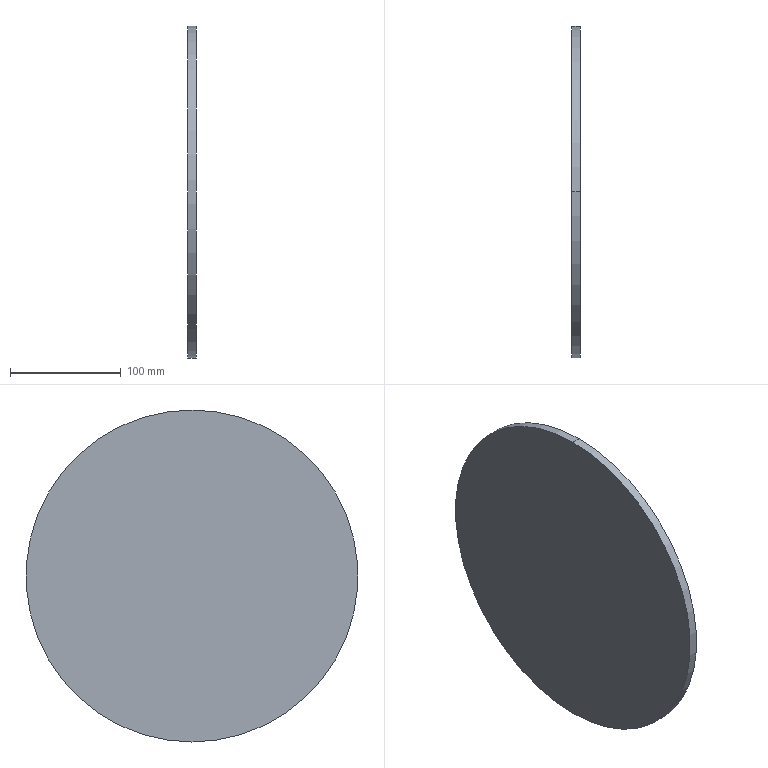Component | SolidWorks | JF21-80.1-1-3(_)-1-SOLID2-1 | 1 solid | 4 faces | box 8 x 300 x 300 mm | volume 565487 mm3 | cylinder 2 | plane 2 | commonest cylinder face diameters 300 x2
STEP:
#1=CARTESIAN_POINT('',(15.433,-39.37,42.126));
#2=VERTEX_POINT('',#1);
#3=CARTESIAN_POINT('',(15.433,-39.37,30.315));
#4=VERTEX_POINT('',#3);
#5=CARTESIAN_POINT('',(15.433,-39.37,36.22));
#6=DIRECTION('',(-1.,0.,0.));
#7=DIRECTION('',(0.,0.,1.));
#8=AXIS2_PLACEMENT_3D('',#5,#6,#7);
#9=CIRCLE('',#8,5.906);
#10=EDGE_CURVE('',#2,#4,#9,.T.);
#11=ORIENTED_EDGE('',*,*,#10,.F.);
#12=CARTESIAN_POINT('',(15.748,-39.37,42.126));
#13=VERTEX_POINT('',#12);
#14=CARTESIAN_POINT('',(15.433,-39.37,42.126));
#15=DIRECTION('',(-1.,0.,0.));
#16=VECTOR('',#15,39.37);
#17=LINE('',#14,#16);
#18=EDGE_CURVE('',#13,#2,#17,.T.);
#19=ORIENTED_EDGE('',*,*,#18,.F.);
#20=CARTESIAN_POINT('',(15.748,-39.37,30.315));
#21=VERTEX_POINT('',#20);
#22=CARTESIAN_POINT('',(15.748,-39.37,36.22));
#23=DIRECTION('',(-1.,0.,0.));
#24=DIRECTION('',(0.,0.,1.));
#25=AXIS2_PLACEMENT_3D('',#22,#23,#24);
#26=CIRCLE('',#25,5.906);
#27=EDGE_CURVE('',#13,#21,#26,.T.);
#28=ORIENTED_EDGE('',*,*,#27,.T.);
#29=CARTESIAN_POINT('',(15.433,-39.37,30.315));
#30=DIRECTION('',(-1.,0.,0.));
#31=VECTOR('',#30,39.37);
#32=LINE('',#29,#31);
#33=EDGE_CURVE('',#21,#4,#32,.T.);
#34=ORIENTED_EDGE('',*,*,#33,.T.);
#35=EDGE_LOOP('',(#11,#19,#28,#34));
#36=FACE_OUTER_BOUND('',#35,.T.);
#37=CARTESIAN_POINT('',(15.433,-39.37,36.22));
#38=DIRECTION('',(1.,0.,0.));
#39=DIRECTION('',(0.,0.,1.));
#40=AXIS2_PLACEMENT_3D('',#37,#38,#39);
#41=CYLINDRICAL_SURFACE('',#40,5.906);
#42=ADVANCED_FACE('',(#36),#41,.T.);
#43=ORIENTED_EDGE('',*,*,#18,.T.);
#44=CARTESIAN_POINT('',(15.433,-39.37,36.22));
#45=DIRECTION('',(-1.,0.,0.));
#46=DIRECTION('',(0.,0.,1.));
#47=AXIS2_PLACEMENT_3D('',#44,#45,#46);
#48=CIRCLE('',#47,5.906);
#49=EDGE_CURVE('',#4,#2,#48,.T.);
#50=ORIENTED_EDGE('',*,*,#49,.F.);
#51=ORIENTED_EDGE('',*,*,#33,.F.);
#52=CARTESIAN_POINT('',(15.748,-39.37,36.22));
#53=DIRECTION('',(-1.,0.,0.));
#54=DIRECTION('',(0.,0.,1.));
#55=AXIS2_PLACEMENT_3D('',#52,#53,#54);
#56=CIRCLE('',#55,5.906);
#57=EDGE_CURVE('',#21,#13,#56,.T.);
#58=ORIENTED_EDGE('',*,*,#57,.T.);
#59=EDGE_LOOP('',(#43,#50,#51,#58));
#60=FACE_OUTER_BOUND('',#59,.T.);
#61=CARTESIAN_POINT('',(15.433,-39.37,36.22));
#62=DIRECTION('',(1.,0.,0.));
#63=DIRECTION('',(0.,0.,1.));
#64=AXIS2_PLACEMENT_3D('',#61,#62,#63);
#65=CYLINDRICAL_SURFACE('',#64,5.906);
#66=ADVANCED_FACE('',(#60),#65,.T.);
#67=ORIENTED_EDGE('',*,*,#49,.T.);
#68=ORIENTED_EDGE('',*,*,#10,.T.);
#69=EDGE_LOOP('',(#67,#68));
#70=FACE_OUTER_BOUND('',#69,.T.);
#71=CARTESIAN_POINT('',(15.433,-39.37,36.22));
#72=DIRECTION('',(-1.,0.,0.));
#73=DIRECTION('',(0.,0.,-1.));
#74=AXIS2_PLACEMENT_3D('',#71,#72,#73);
#75=PLANE('',#74);
#76=ADVANCED_FACE('',(#70),#75,.T.);
#77=ORIENTED_EDGE('',*,*,#57,.F.);
#78=ORIENTED_EDGE('',*,*,#27,.F.);
#79=EDGE_LOOP('',(#77,#78));
#80=FACE_OUTER_BOUND('',#79,.T.);
#81=CARTESIAN_POINT('',(15.748,-39.37,36.22));
#82=DIRECTION('',(-1.,0.,0.));
#83=DIRECTION('',(0.,0.,-1.));
#84=AXIS2_PLACEMENT_3D('',#81,#82,#83);
#85=PLANE('',#84);
#86=ADVANCED_FACE('',(#80),#85,.F.);
#87=CLOSED_SHELL('',(#42,#66,#76,#86));
#88=MANIFOLD_SOLID_BREP('',#87);
#89=CARTESIAN_POINT('',(0.,0.,0.));
#90=DIRECTION('',(0.,0.,1.));
#91=DIRECTION('',(1.,0.,0.));
#92=AXIS2_PLACEMENT_3D('',#89,#90,#91);
#93=(LENGTH_UNIT()NAMED_UNIT(*)SI_UNIT($,.METRE.));
#94=LENGTH_MEASURE_WITH_UNIT(LENGTH_MEASURE(0.0254),#93);
#95=DIMENSIONAL_EXPONENTS(1.,0.,0.,0.,0.,0.,0.);
#96=(CONVERSION_BASED_UNIT('',#94)LENGTH_UNIT()NAMED_UNIT(#95));
#97=UNCERTAINTY_MEASURE_WITH_UNIT(LENGTH_MEASURE(0.00001),#96,'','');
#98=(NAMED_UNIT(*)PLANE_ANGLE_UNIT()SI_UNIT($,.RADIAN.));
#99=(NAMED_UNIT(*)SI_UNIT($,.STERADIAN.)SOLID_ANGLE_UNIT());
#100=(GEOMETRIC_REPRESENTATION_CONTEXT(3)GLOBAL_UNCERTAINTY_ASSIGNED_CONTEXT((#97))GLOBAL_UNIT_ASSIGNED_CONTEXT((#96,#98,#99))REPRESENTATION_CONTEXT('',''));
#101=ADVANCED_BREP_SHAPE_REPRESENTATION('',(#88,#92),#100);
#102=COLOUR_RGB('',0.7922,0.8196,0.9333);
#103=FILL_AREA_STYLE_COLOUR('',#102);
#104=FILL_AREA_STYLE('',(#103));
#105=SURFACE_STYLE_FILL_AREA(#104);
#106=SURFACE_SIDE_STYLE('',(#105));
#107=SURFACE_STYLE_USAGE(.BOTH.,#106);
#108=PRESENTATION_STYLE_ASSIGNMENT((#107));
#109=STYLED_ITEM('',(#108),#88);
#110=PRESENTATION_LAYER_ASSIGNMENT('','',(#109));
#111=(LENGTH_UNIT()NAMED_UNIT(*)SI_UNIT($,.METRE.));
#112=LENGTH_MEASURE_WITH_UNIT(LENGTH_MEASURE(0.0254),#111);
#113=DIMENSIONAL_EXPONENTS(1.,0.,0.,0.,0.,0.,0.);
#114=(CONVERSION_BASED_UNIT('',#112)LENGTH_UNIT()NAMED_UNIT(#113));
#115=UNCERTAINTY_MEASURE_WITH_UNIT(LENGTH_MEASURE(0.00001),#114,'','');
#116=(NAMED_UNIT(*)PLANE_ANGLE_UNIT()SI_UNIT($,.RADIAN.));
#117=(NAMED_UNIT(*)SI_UNIT($,.STERADIAN.)SOLID_ANGLE_UNIT());
#118=(GEOMETRIC_REPRESENTATION_CONTEXT(3)GLOBAL_UNCERTAINTY_ASSIGNED_CONTEXT((#115))GLOBAL_UNIT_ASSIGNED_CONTEXT((#114,#116,#117))REPRESENTATION_CONTEXT('',''));
#119=MECHANICAL_DESIGN_GEOMETRIC_PRESENTATION_REPRESENTATION('',(#109),#118);